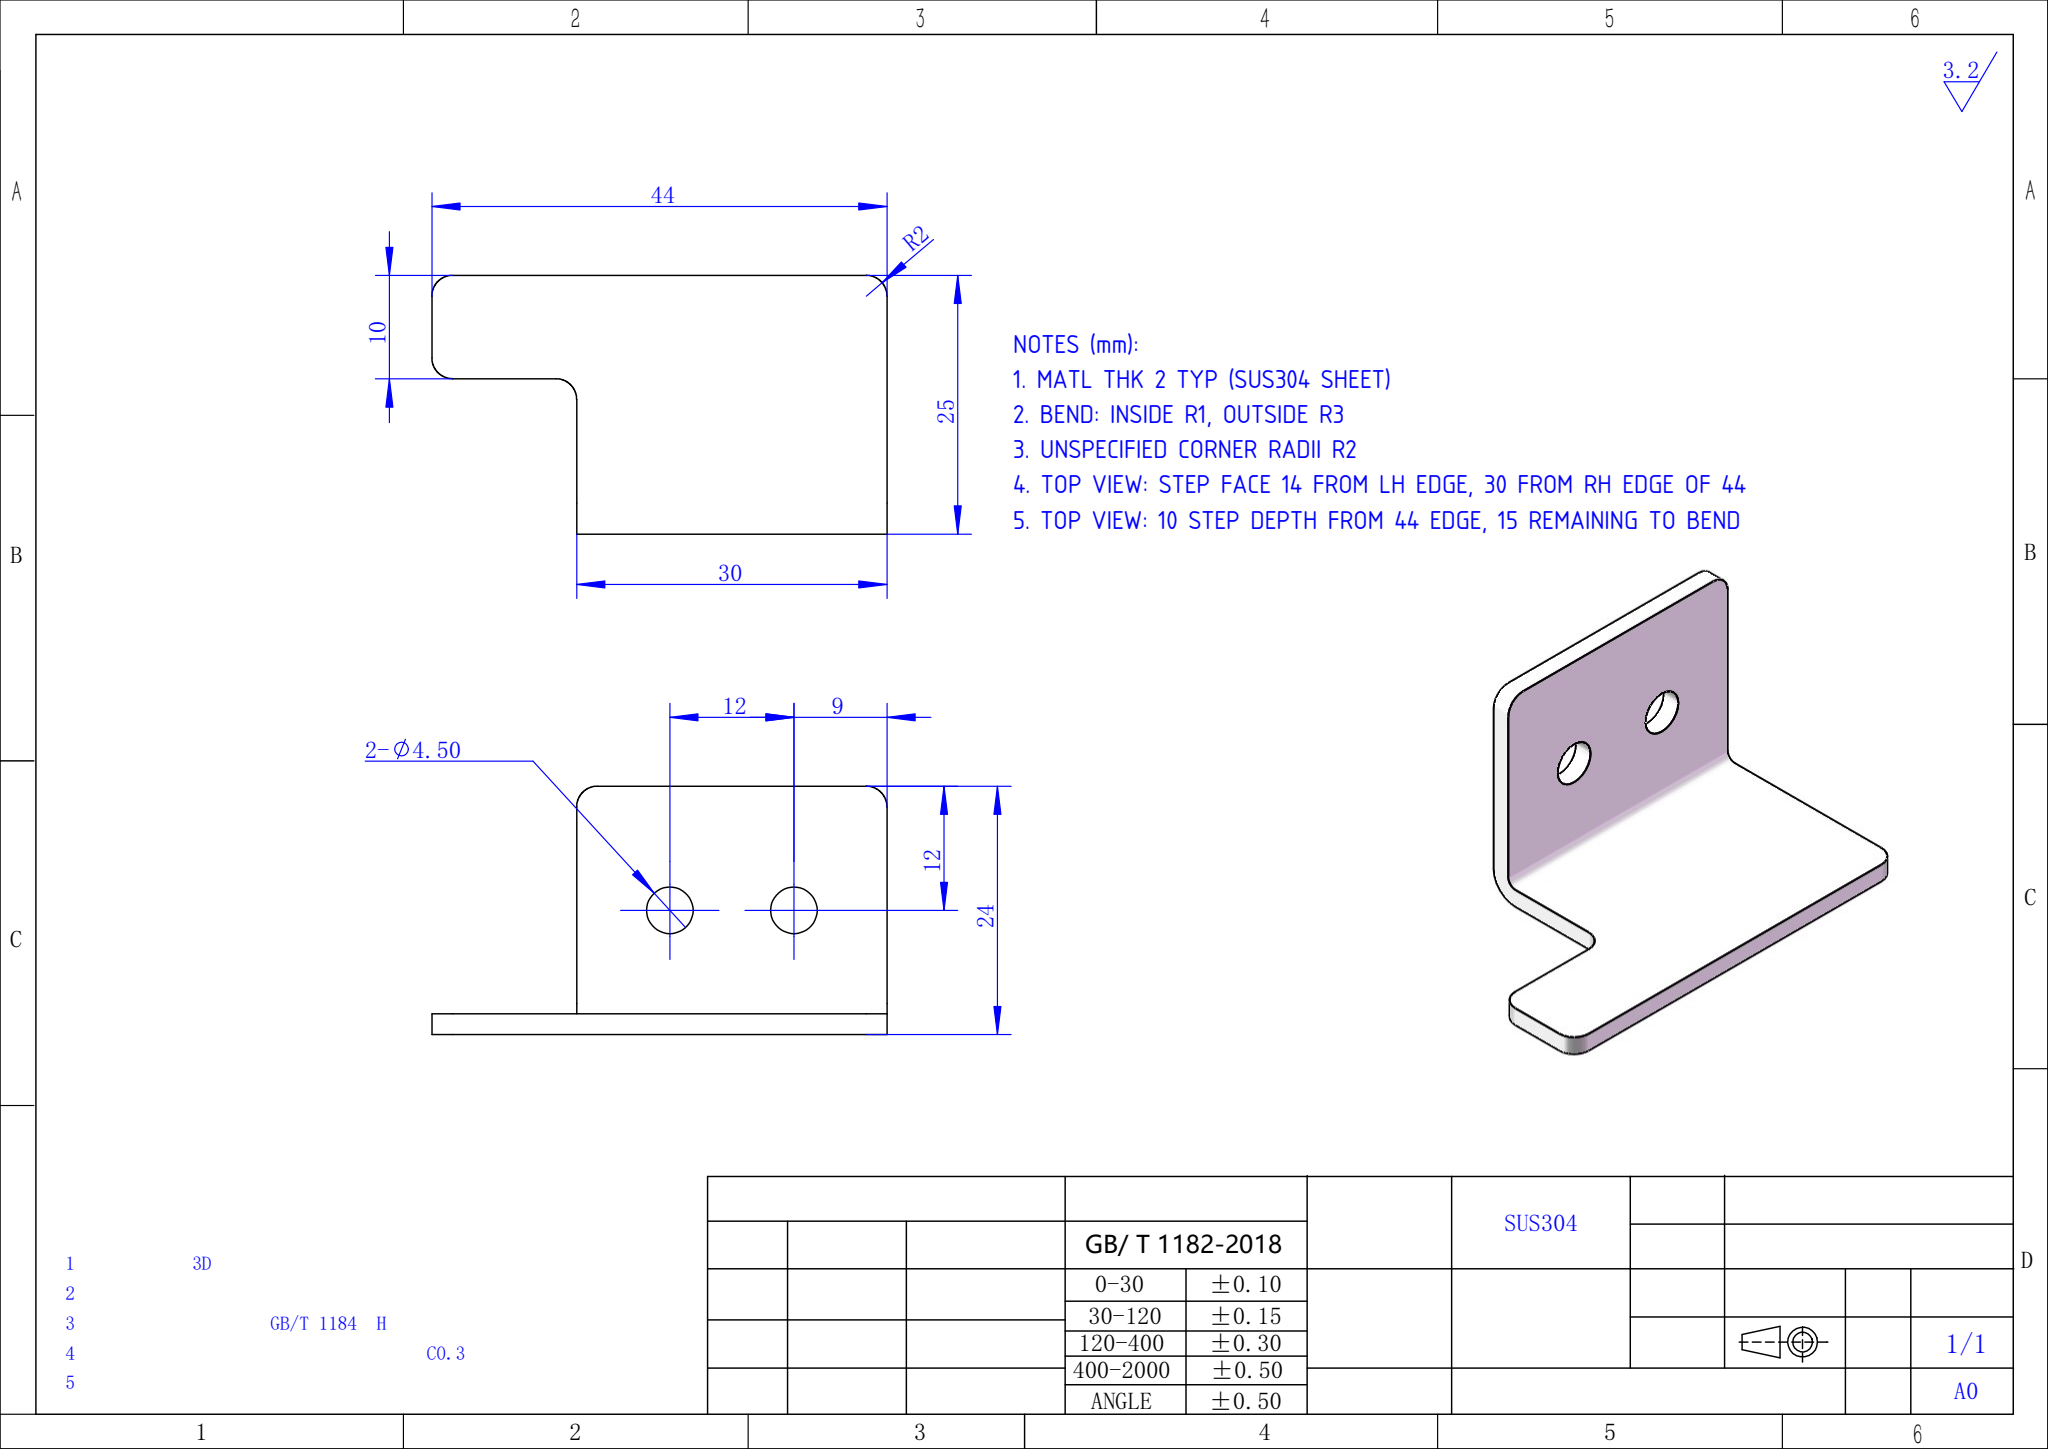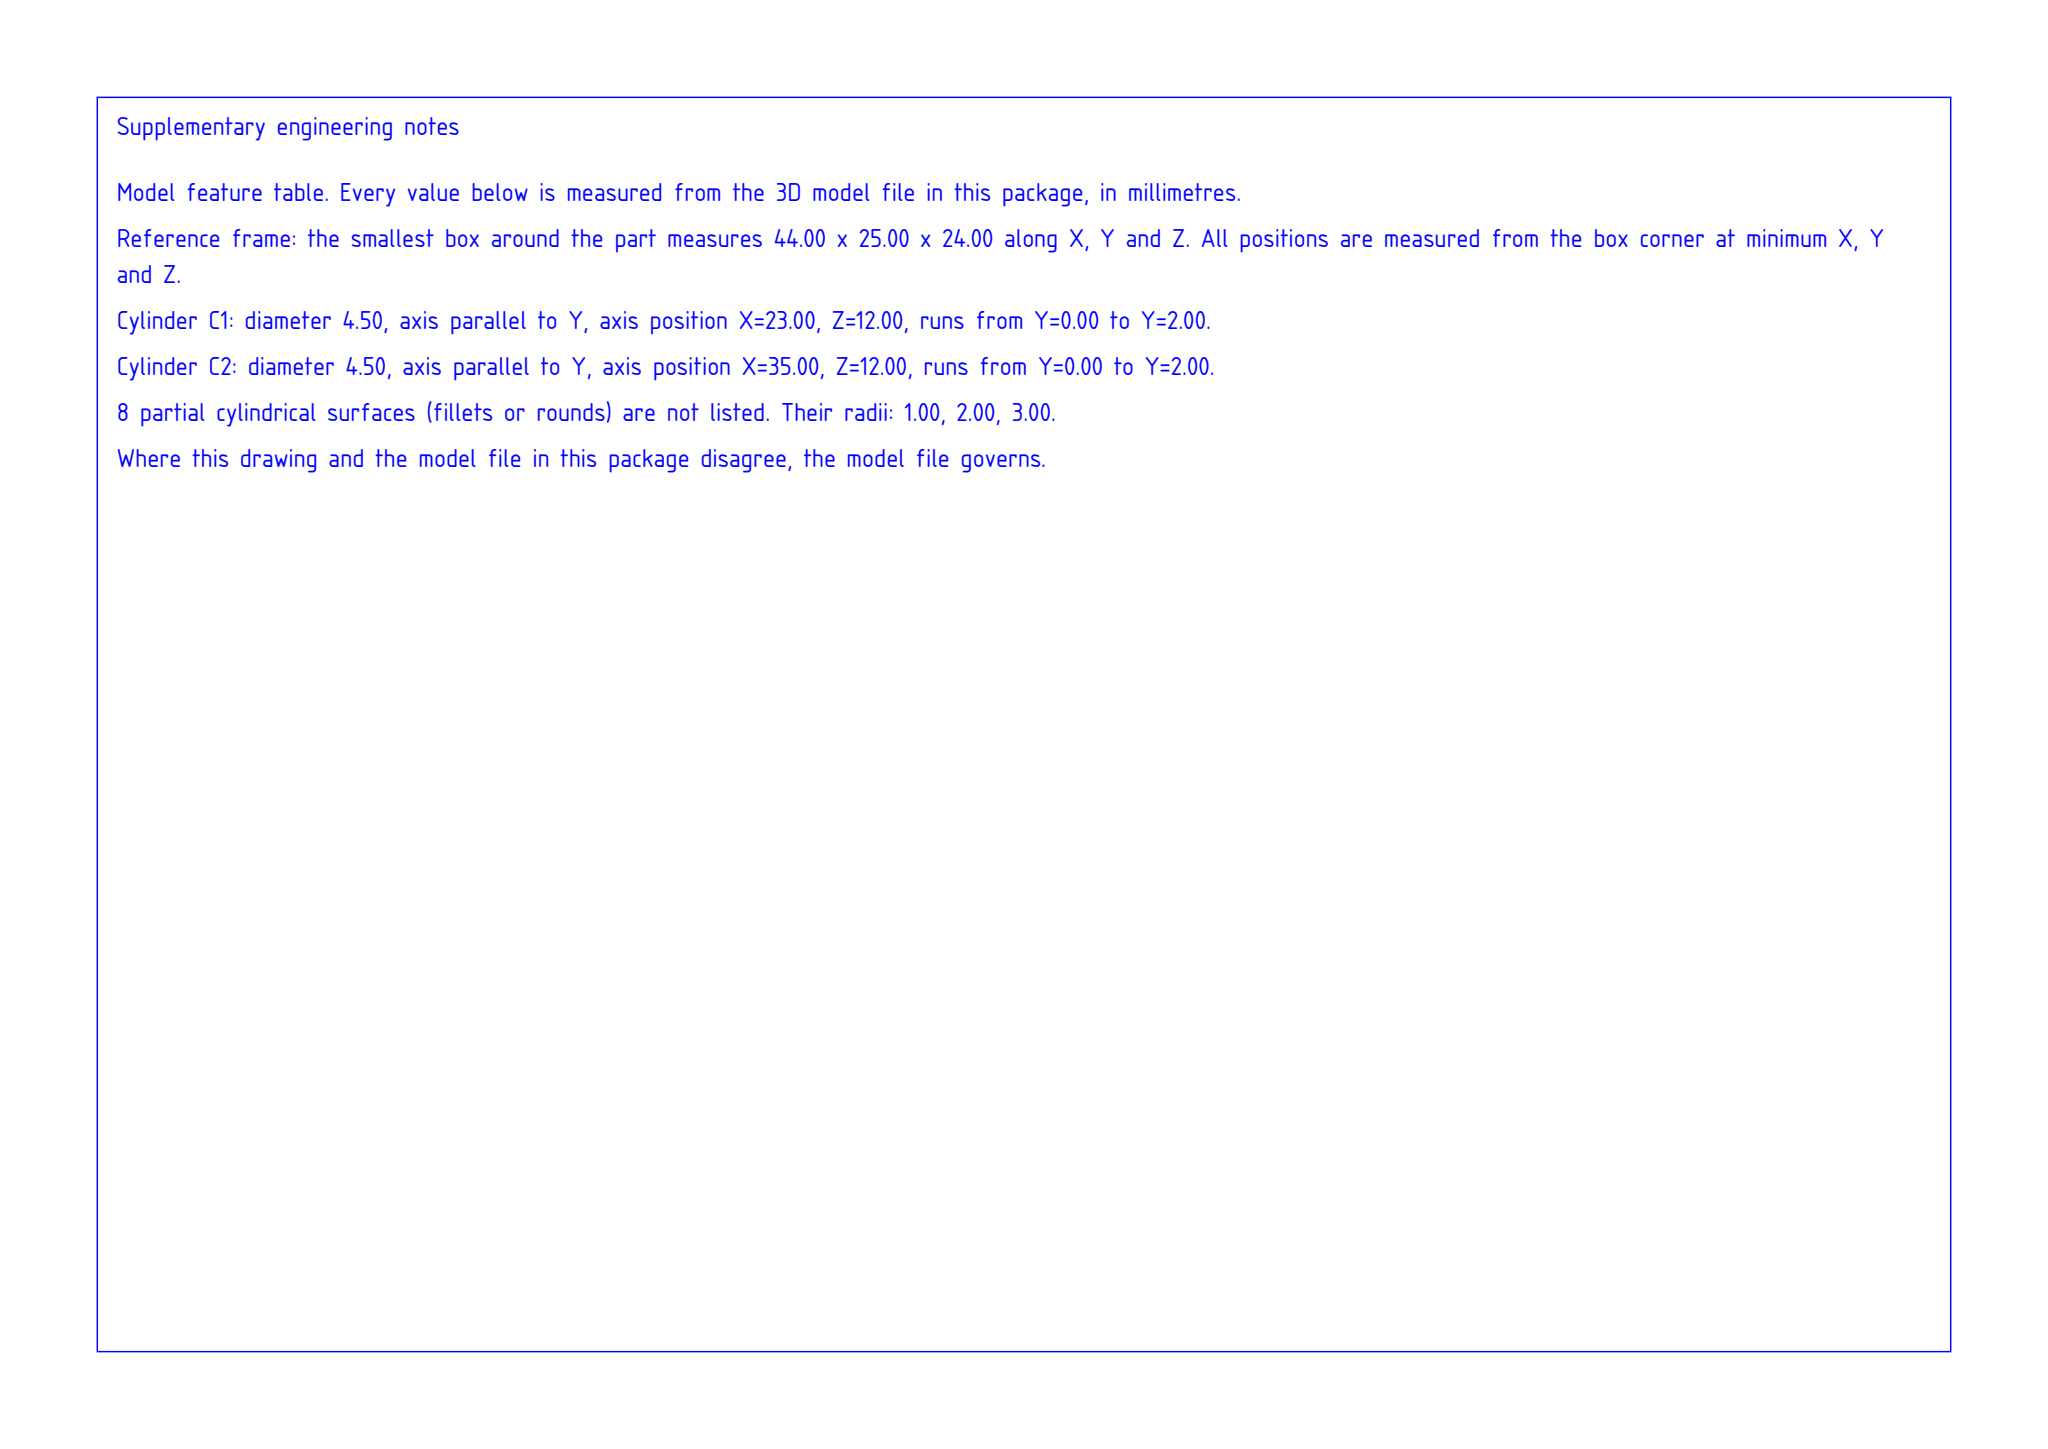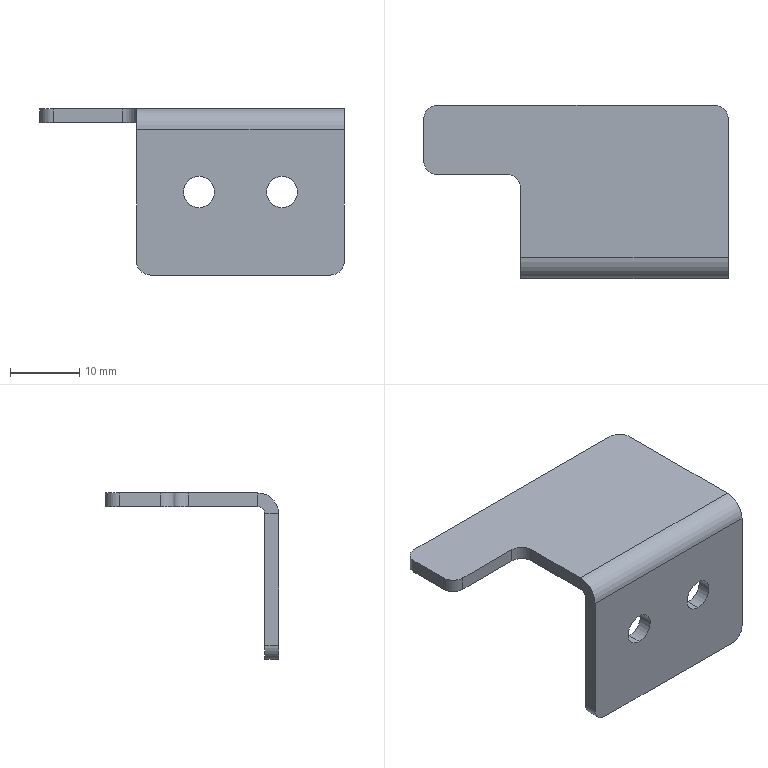Part | SolidWorks | mm | 1 solid | 26 faces | box 44 x 25 x 24 mm | volume 2978 mm3 | plane 14 | cylinder 12 | commonest cylinder face diameters 4 x6 4.5 x4 2 x1 6 x1
Drawing notes:
MATL THK 2 TYP (SUS304 SHEET) | from the solid: Y planes 0 & 2 (horiz plate), Z planes 22 & 24 (vert plate) => 2 mm wall
BEND: INSIDE R1, OUTSIDE R3 | from the solid: X-axis cyls dia 2.0 and dia 6.0 at (y=3,z=21), len 30 = bend inner/outer
UNSPECIFIED CORNER RADII R2 | from the solid: Dia 4.0 vertical/horiz corner cyls at (2,17),(2,23),(12,13),(42,23),(16,2),(42,2)
TOP VIEW: STEP FACE 14 FROM LH EDGE, 30 FROM RH EDGE OF 44 | from the solid: X plane at 14.0 (3 faces) vs bbox X 0-44; 44-14=30 matches 30 dim
TOP VIEW: 10 STEP DEPTH FROM 44 EDGE, 15 REMAINING TO BEND | from the solid: Y plane at 15.0 vs bbox Y 0-25: 25-15=10 strip, 15 remainder
STEP:
#1=CARTESIAN_POINT('',(35.,-2.,-12.25));
#2=VERTEX_POINT('',#1);
#3=CARTESIAN_POINT('',(35.,-2.,-7.75));
#4=VERTEX_POINT('',#3);
#5=CARTESIAN_POINT('',(35.,-2.,-10.));
#6=DIRECTION('',(0.,1.,0.));
#7=DIRECTION('',(0.,0.,1.));
#8=AXIS2_PLACEMENT_3D('',#5,#6,#7);
#9=CIRCLE('',#8,2.25);
#10=EDGE_CURVE('',#2,#4,#9,.T.);
#11=ORIENTED_EDGE('',*,*,#10,.F.);
#12=CARTESIAN_POINT('',(35.,-0.,-12.25));
#13=VERTEX_POINT('',#12);
#14=CARTESIAN_POINT('',(35.,0.,-12.25));
#15=DIRECTION('',(0.,1.,0.));
#16=VECTOR('',#15,1000.);
#17=LINE('',#14,#16);
#18=EDGE_CURVE('',#2,#13,#17,.T.);
#19=ORIENTED_EDGE('',*,*,#18,.T.);
#20=CARTESIAN_POINT('',(35.,-0.,-7.75));
#21=VERTEX_POINT('',#20);
#22=CARTESIAN_POINT('',(35.,-0.,-10.));
#23=DIRECTION('',(0.,1.,0.));
#24=DIRECTION('',(0.,0.,1.));
#25=AXIS2_PLACEMENT_3D('',#22,#23,#24);
#26=CIRCLE('',#25,2.25);
#27=EDGE_CURVE('',#13,#21,#26,.T.);
#28=ORIENTED_EDGE('',*,*,#27,.T.);
#29=CARTESIAN_POINT('',(35.,0.,-7.75));
#30=DIRECTION('',(0.,1.,0.));
#31=VECTOR('',#30,1000.);
#32=LINE('',#29,#31);
#33=EDGE_CURVE('',#4,#21,#32,.T.);
#34=ORIENTED_EDGE('',*,*,#33,.F.);
#35=EDGE_LOOP('',(#11,#19,#28,#34));
#36=FACE_OUTER_BOUND('',#35,.T.);
#37=CARTESIAN_POINT('',(35.,0.,-10.));
#38=DIRECTION('',(0.,1.,0.));
#39=DIRECTION('',(0.,0.,1.));
#40=AXIS2_PLACEMENT_3D('',#37,#38,#39);
#41=CYLINDRICAL_SURFACE('',#40,2.25);
#42=ADVANCED_FACE('',(#36),#41,.F.);
#43=CARTESIAN_POINT('',(23.,-2.,-12.25));
#44=VERTEX_POINT('',#43);
#45=CARTESIAN_POINT('',(23.,-2.,-7.75));
#46=VERTEX_POINT('',#45);
#47=CARTESIAN_POINT('',(23.,-2.,-10.));
#48=DIRECTION('',(0.,1.,0.));
#49=DIRECTION('',(0.,0.,1.));
#50=AXIS2_PLACEMENT_3D('',#47,#48,#49);
#51=CIRCLE('',#50,2.25);
#52=EDGE_CURVE('',#44,#46,#51,.T.);
#53=ORIENTED_EDGE('',*,*,#52,.F.);
#54=CARTESIAN_POINT('',(23.,-0.,-12.25));
#55=VERTEX_POINT('',#54);
#56=CARTESIAN_POINT('',(23.,0.,-12.25));
#57=DIRECTION('',(0.,1.,0.));
#58=VECTOR('',#57,1000.);
#59=LINE('',#56,#58);
#60=EDGE_CURVE('',#44,#55,#59,.T.);
#61=ORIENTED_EDGE('',*,*,#60,.T.);
#62=CARTESIAN_POINT('',(23.,-0.,-7.75));
#63=VERTEX_POINT('',#62);
#64=CARTESIAN_POINT('',(23.,-0.,-10.));
#65=DIRECTION('',(0.,1.,0.));
#66=DIRECTION('',(0.,0.,1.));
#67=AXIS2_PLACEMENT_3D('',#64,#65,#66);
#68=CIRCLE('',#67,2.25);
#69=EDGE_CURVE('',#55,#63,#68,.T.);
#70=ORIENTED_EDGE('',*,*,#69,.T.);
#71=CARTESIAN_POINT('',(23.,0.,-7.75));
#72=DIRECTION('',(0.,1.,0.));
#73=VECTOR('',#72,1000.);
#74=LINE('',#71,#73);
#75=EDGE_CURVE('',#46,#63,#74,.T.);
#76=ORIENTED_EDGE('',*,*,#75,.F.);
#77=EDGE_LOOP('',(#53,#61,#70,#76));
#78=FACE_OUTER_BOUND('',#77,.T.);
#79=CARTESIAN_POINT('',(23.,0.,-10.));
#80=DIRECTION('',(0.,1.,0.));
#81=DIRECTION('',(0.,0.,1.));
#82=AXIS2_PLACEMENT_3D('',#79,#80,#81);
#83=CYLINDRICAL_SURFACE('',#82,2.25);
#84=ADVANCED_FACE('',(#78),#83,.F.);
#85=CARTESIAN_POINT('',(14.,11.,2.));
#86=VERTEX_POINT('',#85);
#87=CARTESIAN_POINT('',(14.,1.,2.));
#88=VERTEX_POINT('',#87);
#89=CARTESIAN_POINT('',(14.,13.,2.));
#90=DIRECTION('',(-0.,-1.,0.));
#91=VECTOR('',#90,1000.);
#92=LINE('',#89,#91);
#93=EDGE_CURVE('',#86,#88,#92,.T.);
#94=ORIENTED_EDGE('',*,*,#93,.F.);
#95=CARTESIAN_POINT('',(14.,11.,0.));
#96=VERTEX_POINT('',#95);
#97=CARTESIAN_POINT('',(14.,11.,0.));
#98=DIRECTION('',(0.,0.,-1.));
#99=VECTOR('',#98,1000.);
#100=LINE('',#97,#99);
#101=EDGE_CURVE('',#86,#96,#100,.T.);
#102=ORIENTED_EDGE('',*,*,#101,.T.);
#103=CARTESIAN_POINT('',(14.,1.,0.));
#104=VERTEX_POINT('',#103);
#105=CARTESIAN_POINT('',(14.,0.,0.));
#106=DIRECTION('',(-0.,-1.,0.));
#107=VECTOR('',#106,1000.);
#108=LINE('',#105,#107);
#109=EDGE_CURVE('',#96,#104,#108,.T.);
#110=ORIENTED_EDGE('',*,*,#109,.T.);
#111=CARTESIAN_POINT('',(14.,1.,0.));
#112=DIRECTION('',(0.,0.,1.));
#113=VECTOR('',#112,1000.);
#114=LINE('',#111,#113);
#115=EDGE_CURVE('',#104,#88,#114,.T.);
#116=ORIENTED_EDGE('',*,*,#115,.T.);
#117=EDGE_LOOP('',(#94,#102,#110,#116));
#118=FACE_OUTER_BOUND('',#117,.T.);
#119=CARTESIAN_POINT('',(14.,13.,2.));
#120=DIRECTION('',(1.,-0.,0.));
#121=DIRECTION('',(0.,1.,0.));
#122=AXIS2_PLACEMENT_3D('',#119,#120,#121);
#123=PLANE('',#122);
#124=ADVANCED_FACE('',(#118),#123,.F.);
#125=CARTESIAN_POINT('',(14.,0.,-1.));
#126=VERTEX_POINT('',#125);
#127=CARTESIAN_POINT('',(14.,0.,-20.));
#128=VERTEX_POINT('',#127);
#129=CARTESIAN_POINT('',(14.,0.,0.));
#130=DIRECTION('',(0.,0.,-1.));
#131=VECTOR('',#130,1000.);
#132=LINE('',#129,#131);
#133=EDGE_CURVE('',#126,#128,#132,.T.);
#134=ORIENTED_EDGE('',*,*,#133,.T.);
#135=CARTESIAN_POINT('',(14.,-2.,-20.));
#136=VERTEX_POINT('',#135);
#137=CARTESIAN_POINT('',(14.,-2.,-20.));
#138=DIRECTION('',(-0.,-1.,0.));
#139=VECTOR('',#138,1000.);
#140=LINE('',#137,#139);
#141=EDGE_CURVE('',#128,#136,#140,.T.);
#142=ORIENTED_EDGE('',*,*,#141,.T.);
#143=CARTESIAN_POINT('',(14.,-2.,-1.));
#144=VERTEX_POINT('',#143);
#145=CARTESIAN_POINT('',(14.,-2.,0.));
#146=DIRECTION('',(0.,0.,-1.));
#147=VECTOR('',#146,1000.);
#148=LINE('',#145,#147);
#149=EDGE_CURVE('',#144,#136,#148,.T.);
#150=ORIENTED_EDGE('',*,*,#149,.F.);
#151=CARTESIAN_POINT('',(14.,-2.,-1.));
#152=DIRECTION('',(0.,1.,0.));
#153=VECTOR('',#152,1000.);
#154=LINE('',#151,#153);
#155=EDGE_CURVE('',#144,#126,#154,.T.);
#156=ORIENTED_EDGE('',*,*,#155,.T.);
#157=EDGE_LOOP('',(#134,#142,#150,#156));
#158=FACE_OUTER_BOUND('',#157,.T.);
#159=CARTESIAN_POINT('',(14.,13.,2.));
#160=DIRECTION('',(1.,-0.,0.));
#161=DIRECTION('',(0.,1.,0.));
#162=AXIS2_PLACEMENT_3D('',#159,#160,#161);
#163=PLANE('',#162);
#164=ADVANCED_FACE('',(#158),#163,.F.);
#165=CARTESIAN_POINT('',(44.,0.,-1.));
#166=VERTEX_POINT('',#165);
#167=CARTESIAN_POINT('',(44.,-2.,-1.));
#168=VERTEX_POINT('',#167);
#169=CARTESIAN_POINT('',(44.,0.,-1.));
#170=DIRECTION('',(0.,-1.,0.));
#171=VECTOR('',#170,1000.);
#172=LINE('',#169,#171);
#173=EDGE_CURVE('',#166,#168,#172,.T.);
#174=ORIENTED_EDGE('',*,*,#173,.F.);
#175=CARTESIAN_POINT('',(44.,1.,0.));
#176=VERTEX_POINT('',#175);
#177=CARTESIAN_POINT('',(44.,1.,-1.));
#178=DIRECTION('',(1.,0.,0.));
#179=DIRECTION('',(0.,0.,1.));
#180=AXIS2_PLACEMENT_3D('',#177,#178,#179);
#181=CIRCLE('',#180,1.);
#182=EDGE_CURVE('',#176,#166,#181,.T.);
#183=ORIENTED_EDGE('',*,*,#182,.F.);
#184=CARTESIAN_POINT('',(44.,1.,2.));
#185=VERTEX_POINT('',#184);
#186=CARTESIAN_POINT('',(44.,1.,2.));
#187=DIRECTION('',(0.,-0.,-1.));
#188=VECTOR('',#187,1000.);
#189=LINE('',#186,#188);
#190=EDGE_CURVE('',#185,#176,#189,.T.);
#191=ORIENTED_EDGE('',*,*,#190,.F.);
#192=CARTESIAN_POINT('',(44.,1.,-1.));
#193=DIRECTION('',(1.,0.,0.));
#194=DIRECTION('',(0.,0.,-1.));
#195=AXIS2_PLACEMENT_3D('',#192,#193,#194);
#196=CIRCLE('',#195,3.);
#197=EDGE_CURVE('',#185,#168,#196,.T.);
#198=ORIENTED_EDGE('',*,*,#197,.T.);
#199=EDGE_LOOP('',(#174,#183,#191,#198));
#200=FACE_OUTER_BOUND('',#199,.T.);
#201=CARTESIAN_POINT('',(44.,0.,-1.));
#202=DIRECTION('',(1.,0.,0.));
#203=DIRECTION('',(0.,0.,-1.));
#204=AXIS2_PLACEMENT_3D('',#201,#202,#203);
#205=PLANE('',#204);
#206=ADVANCED_FACE('',(#200),#205,.T.);
#207=CARTESIAN_POINT('',(44.,-2.,-20.));
#208=VERTEX_POINT('',#207);
#209=CARTESIAN_POINT('',(44.,-2.,0.));
#210=DIRECTION('',(0.,0.,-1.));
#211=VECTOR('',#210,1000.);
#212=LINE('',#209,#211);
#213=EDGE_CURVE('',#168,#208,#212,.T.);
#214=ORIENTED_EDGE('',*,*,#213,.T.);
#215=CARTESIAN_POINT('',(44.,0.,-20.));
#216=VERTEX_POINT('',#215);
#217=CARTESIAN_POINT('',(44.,1.,-20.));
#218=DIRECTION('',(0.,1.,0.));
#219=VECTOR('',#218,1000.);
#220=LINE('',#217,#219);
#221=EDGE_CURVE('',#208,#216,#220,.T.);
#222=ORIENTED_EDGE('',*,*,#221,.T.);
#223=CARTESIAN_POINT('',(44.,0.,0.));
#224=DIRECTION('',(0.,0.,-1.));
#225=VECTOR('',#224,1000.);
#226=LINE('',#223,#225);
#227=EDGE_CURVE('',#166,#216,#226,.T.);
#228=ORIENTED_EDGE('',*,*,#227,.F.);
#229=ORIENTED_EDGE('',*,*,#173,.T.);
#230=EDGE_LOOP('',(#214,#222,#228,#229));
#231=FACE_OUTER_BOUND('',#230,.T.);
#232=CARTESIAN_POINT('',(44.,1.,2.));
#233=DIRECTION('',(1.,0.,0.));
#234=DIRECTION('',(0.,0.,-1.));
#235=AXIS2_PLACEMENT_3D('',#232,#233,#234);
#236=PLANE('',#235);
#237=ADVANCED_FACE('',(#231),#236,.T.);
#238=CARTESIAN_POINT('',(0.,21.,0.));
#239=VERTEX_POINT('',#238);
#240=CARTESIAN_POINT('',(0.,15.,0.));
#241=VERTEX_POINT('',#240);
#242=CARTESIAN_POINT('',(0.,0.,0.));
#243=DIRECTION('',(0.,-1.,0.));
#244=VECTOR('',#243,1000.);
#245=LINE('',#242,#244);
#246=EDGE_CURVE('',#239,#241,#245,.T.);
#247=ORIENTED_EDGE('',*,*,#246,.T.);
#248=CARTESIAN_POINT('',(0.,15.,2.));
#249=VERTEX_POINT('',#248);
#250=CARTESIAN_POINT('',(0.,15.,2.));
#251=DIRECTION('',(0.,0.,1.));
#252=VECTOR('',#251,1000.);
#253=LINE('',#250,#252);
#254=EDGE_CURVE('',#241,#249,#253,.T.);
#255=ORIENTED_EDGE('',*,*,#254,.T.);
#256=CARTESIAN_POINT('',(0.,21.,2.));
#257=VERTEX_POINT('',#256);
#258=CARTESIAN_POINT('',(0.,0.,2.));
#259=DIRECTION('',(0.,-1.,0.));
#260=VECTOR('',#259,1000.);
#261=LINE('',#258,#260);
#262=EDGE_CURVE('',#257,#249,#261,.T.);
#263=ORIENTED_EDGE('',*,*,#262,.F.);
#264=CARTESIAN_POINT('',(0.,21.,-1.));
#265=DIRECTION('',(0.,0.,-1.));
#266=VECTOR('',#265,1000.);
#267=LINE('',#264,#266);
#268=EDGE_CURVE('',#257,#239,#267,.T.);
#269=ORIENTED_EDGE('',*,*,#268,.T.);
#270=EDGE_LOOP('',(#247,#255,#263,#269));
#271=FACE_OUTER_BOUND('',#270,.T.);
#272=CARTESIAN_POINT('',(0.,-2.,-1.));
#273=DIRECTION('',(-1.,0.,0.));
#274=DIRECTION('',(0.,0.,1.));
#275=AXIS2_PLACEMENT_3D('',#272,#273,#274);
#276=PLANE('',#275);
#277=ADVANCED_FACE('',(#271),#276,.T.);
#278=CARTESIAN_POINT('',(35.,-2.,-10.));
#279=DIRECTION('',(0.,1.,0.));
#280=DIRECTION('',(0.,0.,1.));
#281=AXIS2_PLACEMENT_3D('',#278,#279,#280);
#282=CIRCLE('',#281,2.25);
#283=EDGE_CURVE('',#4,#2,#282,.T.);
#284=ORIENTED_EDGE('',*,*,#283,.T.);
#285=ORIENTED_EDGE('',*,*,#10,.T.);
#286=EDGE_LOOP('',(#284,#285));
#287=FACE_BOUND('',#286,.T.);
#288=CARTESIAN_POINT('',(23.,-2.,-10.));
#289=DIRECTION('',(0.,1.,0.));
#290=DIRECTION('',(0.,0.,1.));
#291=AXIS2_PLACEMENT_3D('',#288,#289,#290);
#292=CIRCLE('',#291,2.25);
#293=EDGE_CURVE('',#46,#44,#292,.T.);
#294=ORIENTED_EDGE('',*,*,#293,.T.);
#295=ORIENTED_EDGE('',*,*,#52,.T.);
#296=EDGE_LOOP('',(#294,#295));
#297=FACE_BOUND('',#296,.T.);
#298=CARTESIAN_POINT('',(42.,-2.,-22.));
#299=VERTEX_POINT('',#298);
#300=CARTESIAN_POINT('',(16.,-2.,-22.));
#301=VERTEX_POINT('',#300);
#302=CARTESIAN_POINT('',(44.,-2.,-22.));
#303=DIRECTION('',(-1.,0.,0.));
#304=VECTOR('',#303,1000.);
#305=LINE('',#302,#304);
#306=EDGE_CURVE('',#299,#301,#305,.T.);
#307=ORIENTED_EDGE('',*,*,#306,.F.);
#308=CARTESIAN_POINT('',(42.,-2.,-20.));
#309=DIRECTION('',(0.,-1.,0.));
#310=DIRECTION('',(0.,0.,1.));
#311=AXIS2_PLACEMENT_3D('',#308,#309,#310);
#312=CIRCLE('',#311,2.);
#313=EDGE_CURVE('',#299,#208,#312,.T.);
#314=ORIENTED_EDGE('',*,*,#313,.T.);
#315=ORIENTED_EDGE('',*,*,#213,.F.);
#316=CARTESIAN_POINT('',(44.,-2.,-1.));
#317=DIRECTION('',(-1.,0.,0.));
#318=VECTOR('',#317,1000.);
#319=LINE('',#316,#318);
#320=EDGE_CURVE('',#168,#144,#319,.T.);
#321=ORIENTED_EDGE('',*,*,#320,.T.);
#322=ORIENTED_EDGE('',*,*,#149,.T.);
#323=CARTESIAN_POINT('',(16.,-2.,-20.));
#324=DIRECTION('',(0.,-1.,0.));
#325=DIRECTION('',(0.,0.,1.));
#326=AXIS2_PLACEMENT_3D('',#323,#324,#325);
#327=CIRCLE('',#326,2.);
#328=EDGE_CURVE('',#136,#301,#327,.T.);
#329=ORIENTED_EDGE('',*,*,#328,.T.);
#330=EDGE_LOOP('',(#307,#314,#315,#321,#322,#329));
#331=FACE_OUTER_BOUND('',#330,.T.);
#332=CARTESIAN_POINT('',(44.,-2.,0.));
#333=DIRECTION('',(0.,1.,0.));
#334=DIRECTION('',(0.,0.,1.));
#335=AXIS2_PLACEMENT_3D('',#332,#333,#334);
#336=PLANE('',#335);
#337=ADVANCED_FACE('',(#287,#297,#331),#336,.F.);
#338=CARTESIAN_POINT('',(42.,0.,-22.));
#339=VERTEX_POINT('',#338);
#340=CARTESIAN_POINT('',(16.,0.,-22.));
#341=VERTEX_POINT('',#340);
#342=CARTESIAN_POINT('',(44.,0.,-22.));
#343=DIRECTION('',(-1.,0.,0.));
#344=VECTOR('',#343,1000.);
#345=LINE('',#342,#344);
#346=EDGE_CURVE('',#339,#341,#345,.T.);
#347=ORIENTED_EDGE('',*,*,#346,.F.);
#348=CARTESIAN_POINT('',(42.,0.,-22.));
#349=DIRECTION('',(0.,-1.,0.));
#350=VECTOR('',#349,1000.);
#351=LINE('',#348,#350);
#352=EDGE_CURVE('',#339,#299,#351,.T.);
#353=ORIENTED_EDGE('',*,*,#352,.T.);
#354=ORIENTED_EDGE('',*,*,#306,.T.);
#355=CARTESIAN_POINT('',(16.,0.,-22.));
#356=DIRECTION('',(0.,1.,0.));
#357=VECTOR('',#356,1000.);
#358=LINE('',#355,#357);
#359=EDGE_CURVE('',#301,#341,#358,.T.);
#360=ORIENTED_EDGE('',*,*,#359,.T.);
#361=EDGE_LOOP('',(#347,#353,#354,#360));
#362=FACE_OUTER_BOUND('',#361,.T.);
#363=CARTESIAN_POINT('',(44.,0.,-22.));
#364=DIRECTION('',(0.,0.,-1.));
#365=DIRECTION('',(-1.,0.,0.));
#366=AXIS2_PLACEMENT_3D('',#363,#364,#365);
#367=PLANE('',#366);
#368=ADVANCED_FACE('',(#362),#367,.T.);
#369=CARTESIAN_POINT('',(35.,-0.,-10.));
#370=DIRECTION('',(0.,1.,0.));
#371=DIRECTION('',(0.,0.,1.));
#372=AXIS2_PLACEMENT_3D('',#369,#370,#371);
#373=CIRCLE('',#372,2.25);
#374=EDGE_CURVE('',#21,#13,#373,.T.);
#375=ORIENTED_EDGE('',*,*,#374,.F.);
#376=ORIENTED_EDGE('',*,*,#27,.F.);
#377=EDGE_LOOP('',(#375,#376));
#378=FACE_BOUND('',#377,.T.);
#379=CARTESIAN_POINT('',(23.,-0.,-10.));
#380=DIRECTION('',(0.,1.,0.));
#381=DIRECTION('',(0.,0.,1.));
#382=AXIS2_PLACEMENT_3D('',#379,#380,#381);
#383=CIRCLE('',#382,2.25);
#384=EDGE_CURVE('',#63,#55,#383,.T.);
#385=ORIENTED_EDGE('',*,*,#384,.F.);
#386=ORIENTED_EDGE('',*,*,#69,.F.);
#387=EDGE_LOOP('',(#385,#386));
#388=FACE_BOUND('',#387,.T.);
#389=ORIENTED_EDGE('',*,*,#227,.T.);
#390=CARTESIAN_POINT('',(42.,0.,-20.));
#391=DIRECTION('',(0.,1.,0.));
#392=DIRECTION('',(0.,0.,1.));
#393=AXIS2_PLACEMENT_3D('',#390,#391,#392);
#394=CIRCLE('',#393,2.);
#395=EDGE_CURVE('',#216,#339,#394,.T.);
#396=ORIENTED_EDGE('',*,*,#395,.T.);
#397=ORIENTED_EDGE('',*,*,#346,.T.);
#398=CARTESIAN_POINT('',(16.,0.,-20.));
#399=DIRECTION('',(0.,1.,0.));
#400=DIRECTION('',(0.,0.,1.));
#401=AXIS2_PLACEMENT_3D('',#398,#399,#400);
#402=CIRCLE('',#401,2.);
#403=EDGE_CURVE('',#341,#128,#402,.T.);
#404=ORIENTED_EDGE('',*,*,#403,.T.);
#405=ORIENTED_EDGE('',*,*,#133,.F.);
#406=CARTESIAN_POINT('',(44.,0.,-1.));
#407=DIRECTION('',(-1.,0.,0.));
#408=VECTOR('',#407,1000.);
#409=LINE('',#406,#408);
#410=EDGE_CURVE('',#166,#126,#409,.T.);
#411=ORIENTED_EDGE('',*,*,#410,.F.);
#412=EDGE_LOOP('',(#389,#396,#397,#404,#405,#411));
#413=FACE_OUTER_BOUND('',#412,.T.);
#414=CARTESIAN_POINT('',(44.,0.,0.));
#415=DIRECTION('',(0.,1.,0.));
#416=DIRECTION('',(0.,0.,1.));
#417=AXIS2_PLACEMENT_3D('',#414,#415,#416);
#418=PLANE('',#417);
#419=ADVANCED_FACE('',(#378,#388,#413),#418,.T.);
#420=CARTESIAN_POINT('',(14.,1.,-1.));
#421=DIRECTION('',(1.,-0.,0.));
#422=DIRECTION('',(0.,1.,0.));
#423=AXIS2_PLACEMENT_3D('',#420,#421,#422);
#424=CIRCLE('',#423,1.);
#425=EDGE_CURVE('',#104,#126,#424,.T.);
#426=ORIENTED_EDGE('',*,*,#425,.F.);
#427=CARTESIAN_POINT('',(44.,1.,0.));
#428=DIRECTION('',(-1.,0.,0.));
#429=VECTOR('',#428,1000.);
#430=LINE('',#427,#429);
#431=EDGE_CURVE('',#176,#104,#430,.T.);
#432=ORIENTED_EDGE('',*,*,#431,.F.);
#433=ORIENTED_EDGE('',*,*,#182,.T.);
#434=ORIENTED_EDGE('',*,*,#410,.T.);
#435=EDGE_LOOP('',(#426,#432,#433,#434));
#436=FACE_OUTER_BOUND('',#435,.T.);
#437=CARTESIAN_POINT('',(44.,1.,-1.));
#438=DIRECTION('',(-1.,0.,0.));
#439=DIRECTION('',(0.,0.,1.));
#440=AXIS2_PLACEMENT_3D('',#437,#438,#439);
#441=CYLINDRICAL_SURFACE('',#440,1.);
#442=ADVANCED_FACE('',(#436),#441,.F.);
#443=CARTESIAN_POINT('',(2.,13.,0.));
#444=VERTEX_POINT('',#443);
#445=CARTESIAN_POINT('',(12.,13.,0.));
#446=VERTEX_POINT('',#445);
#447=CARTESIAN_POINT('',(44.,13.,0.));
#448=DIRECTION('',(1.,0.,0.));
#449=VECTOR('',#448,1000.);
#450=LINE('',#447,#449);
#451=EDGE_CURVE('',#444,#446,#450,.T.);
#452=ORIENTED_EDGE('',*,*,#451,.F.);
#453=CARTESIAN_POINT('',(2.,15.,0.));
#454=DIRECTION('',(0.,0.,-1.));
#455=DIRECTION('',(-1.,0.,0.));
#456=AXIS2_PLACEMENT_3D('',#453,#454,#455);
#457=CIRCLE('',#456,2.);
#458=EDGE_CURVE('',#444,#241,#457,.T.);
#459=ORIENTED_EDGE('',*,*,#458,.T.);
#460=ORIENTED_EDGE('',*,*,#246,.F.);
#461=CARTESIAN_POINT('',(2.,23.,0.));
#462=VERTEX_POINT('',#461);
#463=CARTESIAN_POINT('',(2.,21.,0.));
#464=DIRECTION('',(0.,0.,-1.));
#465=DIRECTION('',(-1.,0.,0.));
#466=AXIS2_PLACEMENT_3D('',#463,#464,#465);
#467=CIRCLE('',#466,2.);
#468=EDGE_CURVE('',#239,#462,#467,.T.);
#469=ORIENTED_EDGE('',*,*,#468,.T.);
#470=CARTESIAN_POINT('',(42.,23.,0.));
#471=VERTEX_POINT('',#470);
#472=CARTESIAN_POINT('',(44.,23.,0.));
#473=DIRECTION('',(-1.,0.,0.));
#474=VECTOR('',#473,1000.);
#475=LINE('',#472,#474);
#476=EDGE_CURVE('',#471,#462,#475,.T.);
#477=ORIENTED_EDGE('',*,*,#476,.F.);
#478=CARTESIAN_POINT('',(44.,21.,0.));
#479=VERTEX_POINT('',#478);
#480=CARTESIAN_POINT('',(42.,21.,0.));
#481=DIRECTION('',(0.,0.,-1.));
#482=DIRECTION('',(-1.,0.,0.));
#483=AXIS2_PLACEMENT_3D('',#480,#481,#482);
#484=CIRCLE('',#483,2.);
#485=EDGE_CURVE('',#471,#479,#484,.T.);
#486=ORIENTED_EDGE('',*,*,#485,.T.);
#487=CARTESIAN_POINT('',(44.,0.,0.));
#488=DIRECTION('',(0.,-1.,0.));
#489=VECTOR('',#488,1000.);
#490=LINE('',#487,#489);
#491=EDGE_CURVE('',#479,#176,#490,.T.);
#492=ORIENTED_EDGE('',*,*,#491,.T.);
#493=ORIENTED_EDGE('',*,*,#431,.T.);
#494=ORIENTED_EDGE('',*,*,#109,.F.);
#495=CARTESIAN_POINT('',(12.,11.,0.));
#496=DIRECTION('',(0.,0.,1.));
#497=DIRECTION('',(-1.,0.,0.));
#498=AXIS2_PLACEMENT_3D('',#495,#496,#497);
#499=CIRCLE('',#498,2.);
#500=EDGE_CURVE('',#96,#446,#499,.T.);
#501=ORIENTED_EDGE('',*,*,#500,.T.);
#502=EDGE_LOOP('',(#452,#459,#460,#469,#477,#486,#492,#493,#494,#501));
#503=FACE_OUTER_BOUND('',#502,.T.);
#504=CARTESIAN_POINT('',(44.,0.,0.));
#505=DIRECTION('',(0.,0.,-1.));
#506=DIRECTION('',(-1.,0.,0.));
#507=AXIS2_PLACEMENT_3D('',#504,#505,#506);
#508=PLANE('',#507);
#509=ADVANCED_FACE('',(#503),#508,.T.);
#510=ORIENTED_EDGE('',*,*,#476,.T.);
#511=CARTESIAN_POINT('',(2.,23.,2.));
#512=VERTEX_POINT('',#511);
#513=CARTESIAN_POINT('',(2.,23.,2.));
#514=DIRECTION('',(0.,0.,1.));
#515=VECTOR('',#514,1000.);
#516=LINE('',#513,#515);
#517=EDGE_CURVE('',#462,#512,#516,.T.);
#518=ORIENTED_EDGE('',*,*,#517,.T.);
#519=CARTESIAN_POINT('',(42.,23.,2.));
#520=VERTEX_POINT('',#519);
#521=CARTESIAN_POINT('',(44.,23.,2.));
#522=DIRECTION('',(-1.,0.,0.));
#523=VECTOR('',#522,1000.);
#524=LINE('',#521,#523);
#525=EDGE_CURVE('',#520,#512,#524,.T.);
#526=ORIENTED_EDGE('',*,*,#525,.F.);
#527=CARTESIAN_POINT('',(42.,23.,0.));
#528=DIRECTION('',(0.,0.,-1.));
#529=VECTOR('',#528,1000.);
#530=LINE('',#527,#529);
#531=EDGE_CURVE('',#520,#471,#530,.T.);
#532=ORIENTED_EDGE('',*,*,#531,.T.);
#533=EDGE_LOOP('',(#510,#518,#526,#532));
#534=FACE_OUTER_BOUND('',#533,.T.);
#535=CARTESIAN_POINT('',(44.,23.,2.));
#536=DIRECTION('',(0.,1.,0.));
#537=DIRECTION('',(0.,0.,1.));
#538=AXIS2_PLACEMENT_3D('',#535,#536,#537);
#539=PLANE('',#538);
#540=ADVANCED_FACE('',(#534),#539,.T.);
#541=ORIENTED_EDGE('',*,*,#262,.T.);
#542=CARTESIAN_POINT('',(2.,13.,2.));
#543=VERTEX_POINT('',#542);
#544=CARTESIAN_POINT('',(2.,15.,2.));
#545=DIRECTION('',(0.,0.,1.));
#546=DIRECTION('',(-1.,0.,0.));
#547=AXIS2_PLACEMENT_3D('',#544,#545,#546);
#548=CIRCLE('',#547,2.);
#549=EDGE_CURVE('',#249,#543,#548,.T.);
#550=ORIENTED_EDGE('',*,*,#549,.T.);
#551=CARTESIAN_POINT('',(12.,13.,2.));
#552=VERTEX_POINT('',#551);
#553=CARTESIAN_POINT('',(14.,13.,2.));
#554=DIRECTION('',(1.,0.,0.));
#555=VECTOR('',#554,1000.);
#556=LINE('',#553,#555);
#557=EDGE_CURVE('',#543,#552,#556,.T.);
#558=ORIENTED_EDGE('',*,*,#557,.T.);
#559=CARTESIAN_POINT('',(12.,11.,2.));
#560=DIRECTION('',(0.,0.,-1.));
#561=DIRECTION('',(-1.,0.,0.));
#562=AXIS2_PLACEMENT_3D('',#559,#560,#561);
#563=CIRCLE('',#562,2.);
#564=EDGE_CURVE('',#552,#86,#563,.T.);
#565=ORIENTED_EDGE('',*,*,#564,.T.);
#566=ORIENTED_EDGE('',*,*,#93,.T.);
#567=CARTESIAN_POINT('',(44.,1.,2.));
#568=DIRECTION('',(-1.,0.,0.));
#569=VECTOR('',#568,1000.);
#570=LINE('',#567,#569);
#571=EDGE_CURVE('',#185,#88,#570,.T.);
#572=ORIENTED_EDGE('',*,*,#571,.F.);
#573=CARTESIAN_POINT('',(44.,21.,2.));
#574=VERTEX_POINT('',#573);
#575=CARTESIAN_POINT('',(44.,0.,2.));
#576=DIRECTION('',(0.,-1.,0.));
#577=VECTOR('',#576,1000.);
#578=LINE('',#575,#577);
#579=EDGE_CURVE('',#574,#185,#578,.T.);
#580=ORIENTED_EDGE('',*,*,#579,.F.);
#581=CARTESIAN_POINT('',(42.,21.,2.));
#582=DIRECTION('',(0.,0.,1.));
#583=DIRECTION('',(-1.,0.,0.));
#584=AXIS2_PLACEMENT_3D('',#581,#582,#583);
#585=CIRCLE('',#584,2.);
#586=EDGE_CURVE('',#574,#520,#585,.T.);
#587=ORIENTED_EDGE('',*,*,#586,.T.);
#588=ORIENTED_EDGE('',*,*,#525,.T.);
#589=CARTESIAN_POINT('',(2.,21.,2.));
#590=DIRECTION('',(0.,0.,1.));
#591=DIRECTION('',(-1.,0.,0.));
#592=AXIS2_PLACEMENT_3D('',#589,#590,#591);
#593=CIRCLE('',#592,2.);
#594=EDGE_CURVE('',#512,#257,#593,.T.);
#595=ORIENTED_EDGE('',*,*,#594,.T.);
#596=EDGE_LOOP('',(#541,#550,#558,#565,#566,#572,#580,#587,#588,#595));
#597=FACE_OUTER_BOUND('',#596,.T.);
#598=CARTESIAN_POINT('',(44.,0.,2.));
#599=DIRECTION('',(0.,0.,-1.));
#600=DIRECTION('',(-1.,0.,0.));
#601=AXIS2_PLACEMENT_3D('',#598,#599,#600);
#602=PLANE('',#601);
#603=ADVANCED_FACE('',(#597),#602,.F.);
#604=ORIENTED_EDGE('',*,*,#571,.T.);
#605=CARTESIAN_POINT('',(14.,1.,-1.));
#606=DIRECTION('',(1.,-0.,0.));
#607=DIRECTION('',(0.,1.,0.));
#608=AXIS2_PLACEMENT_3D('',#605,#606,#607);
#609=CIRCLE('',#608,3.);
#610=EDGE_CURVE('',#88,#144,#609,.T.);
#611=ORIENTED_EDGE('',*,*,#610,.T.);
#612=ORIENTED_EDGE('',*,*,#320,.F.);
#613=ORIENTED_EDGE('',*,*,#197,.F.);
#614=EDGE_LOOP('',(#604,#611,#612,#613));
#615=FACE_OUTER_BOUND('',#614,.T.);
#616=CARTESIAN_POINT('',(44.,1.,-1.));
#617=DIRECTION('',(-1.,0.,0.));
#618=DIRECTION('',(0.,0.,1.));
#619=AXIS2_PLACEMENT_3D('',#616,#617,#618);
#620=CYLINDRICAL_SURFACE('',#619,3.);
#621=ADVANCED_FACE('',(#615),#620,.T.);
#622=ORIENTED_EDGE('',*,*,#491,.F.);
#623=CARTESIAN_POINT('',(44.,21.,2.));
#624=DIRECTION('',(0.,0.,1.));
#625=VECTOR('',#624,1000.);
#626=LINE('',#623,#625);
#627=EDGE_CURVE('',#479,#574,#626,.T.);
#628=ORIENTED_EDGE('',*,*,#627,.T.);
#629=ORIENTED_EDGE('',*,*,#579,.T.);
#630=ORIENTED_EDGE('',*,*,#190,.T.);
#631=EDGE_LOOP('',(#622,#628,#629,#630));
#632=FACE_OUTER_BOUND('',#631,.T.);
#633=CARTESIAN_POINT('',(44.,1.,-1.));
#634=DIRECTION('',(-1.,0.,0.));
#635=DIRECTION('',(0.,0.,1.));
#636=AXIS2_PLACEMENT_3D('',#633,#634,#635);
#637=PLANE('',#636);
#638=ADVANCED_FACE('',(#632),#637,.F.);
#639=ORIENTED_EDGE('',*,*,#115,.F.);
#640=ORIENTED_EDGE('',*,*,#425,.T.);
#641=ORIENTED_EDGE('',*,*,#155,.F.);
#642=ORIENTED_EDGE('',*,*,#610,.F.);
#643=EDGE_LOOP('',(#639,#640,#641,#642));
#644=FACE_OUTER_BOUND('',#643,.T.);
#645=CARTESIAN_POINT('',(14.,13.,2.));
#646=DIRECTION('',(1.,-0.,0.));
#647=DIRECTION('',(0.,1.,0.));
#648=AXIS2_PLACEMENT_3D('',#645,#646,#647);
#649=PLANE('',#648);
#650=ADVANCED_FACE('',(#644),#649,.F.);
#651=ORIENTED_EDGE('',*,*,#451,.T.);
#652=CARTESIAN_POINT('',(12.,13.,2.));
#653=DIRECTION('',(0.,0.,1.));
#654=VECTOR('',#653,1000.);
#655=LINE('',#652,#654);
#656=EDGE_CURVE('',#446,#552,#655,.T.);
#657=ORIENTED_EDGE('',*,*,#656,.T.);
#658=ORIENTED_EDGE('',*,*,#557,.F.);
#659=CARTESIAN_POINT('',(2.,13.,0.));
#660=DIRECTION('',(0.,0.,-1.));
#661=VECTOR('',#660,1000.);
#662=LINE('',#659,#661);
#663=EDGE_CURVE('',#543,#444,#662,.T.);
#664=ORIENTED_EDGE('',*,*,#663,.T.);
#665=EDGE_LOOP('',(#651,#657,#658,#664));
#666=FACE_OUTER_BOUND('',#665,.T.);
#667=CARTESIAN_POINT('',(14.,13.,2.));
#668=DIRECTION('',(0.,1.,0.));
#669=DIRECTION('',(0.,0.,1.));
#670=AXIS2_PLACEMENT_3D('',#667,#668,#669);
#671=PLANE('',#670);
#672=ADVANCED_FACE('',(#666),#671,.F.);
#673=ORIENTED_EDGE('',*,*,#564,.F.);
#674=ORIENTED_EDGE('',*,*,#656,.F.);
#675=ORIENTED_EDGE('',*,*,#500,.F.);
#676=ORIENTED_EDGE('',*,*,#101,.F.);
#677=EDGE_LOOP('',(#673,#674,#675,#676));
#678=FACE_OUTER_BOUND('',#677,.T.);
#679=CARTESIAN_POINT('',(12.,11.,2.));
#680=DIRECTION('',(0.,0.,1.));
#681=DIRECTION('',(1.,0.,0.));
#682=AXIS2_PLACEMENT_3D('',#679,#680,#681);
#683=CYLINDRICAL_SURFACE('',#682,2.);
#684=ADVANCED_FACE('',(#678),#683,.F.);
#685=ORIENTED_EDGE('',*,*,#395,.F.);
#686=ORIENTED_EDGE('',*,*,#221,.F.);
#687=ORIENTED_EDGE('',*,*,#313,.F.);
#688=ORIENTED_EDGE('',*,*,#352,.F.);
#689=EDGE_LOOP('',(#685,#686,#687,#688));
#690=FACE_OUTER_BOUND('',#689,.T.);
#691=CARTESIAN_POINT('',(42.,0.,-20.));
#692=DIRECTION('',(0.,-1.,0.));
#693=DIRECTION('',(0.,0.,-1.));
#694=AXIS2_PLACEMENT_3D('',#691,#692,#693);
#695=CYLINDRICAL_SURFACE('',#694,2.);
#696=ADVANCED_FACE('',(#690),#695,.T.);
#697=ORIENTED_EDGE('',*,*,#403,.F.);
#698=ORIENTED_EDGE('',*,*,#359,.F.);
#699=ORIENTED_EDGE('',*,*,#328,.F.);
#700=ORIENTED_EDGE('',*,*,#141,.F.);
#701=EDGE_LOOP('',(#697,#698,#699,#700));
#702=FACE_OUTER_BOUND('',#701,.T.);
#703=CARTESIAN_POINT('',(16.,13.,-20.));
#704=DIRECTION('',(0.,1.,0.));
#705=DIRECTION('',(-1.,0.,0.));
#706=AXIS2_PLACEMENT_3D('',#703,#704,#705);
#707=CYLINDRICAL_SURFACE('',#706,2.);
#708=ADVANCED_FACE('',(#702),#707,.T.);
#709=ORIENTED_EDGE('',*,*,#549,.F.);
#710=ORIENTED_EDGE('',*,*,#254,.F.);
#711=ORIENTED_EDGE('',*,*,#458,.F.);
#712=ORIENTED_EDGE('',*,*,#663,.F.);
#713=EDGE_LOOP('',(#709,#710,#711,#712));
#714=FACE_OUTER_BOUND('',#713,.T.);
#715=CARTESIAN_POINT('',(2.,15.,2.));
#716=DIRECTION('',(0.,0.,1.));
#717=DIRECTION('',(1.,0.,0.));
#718=AXIS2_PLACEMENT_3D('',#715,#716,#717);
#719=CYLINDRICAL_SURFACE('',#718,2.);
#720=ADVANCED_FACE('',(#714),#719,.T.);
#721=ORIENTED_EDGE('',*,*,#594,.F.);
#722=ORIENTED_EDGE('',*,*,#517,.F.);
#723=ORIENTED_EDGE('',*,*,#468,.F.);
#724=ORIENTED_EDGE('',*,*,#268,.F.);
#725=EDGE_LOOP('',(#721,#722,#723,#724));
#726=FACE_OUTER_BOUND('',#725,.T.);
#727=CARTESIAN_POINT('',(2.,21.,-1.));
#728=DIRECTION('',(0.,0.,-1.));
#729=DIRECTION('',(-1.,0.,0.));
#730=AXIS2_PLACEMENT_3D('',#727,#728,#729);
#731=CYLINDRICAL_SURFACE('',#730,2.);
#732=ADVANCED_FACE('',(#726),#731,.T.);
#733=ORIENTED_EDGE('',*,*,#586,.F.);
#734=ORIENTED_EDGE('',*,*,#627,.F.);
#735=ORIENTED_EDGE('',*,*,#485,.F.);
#736=ORIENTED_EDGE('',*,*,#531,.F.);
#737=EDGE_LOOP('',(#733,#734,#735,#736));
#738=FACE_OUTER_BOUND('',#737,.T.);
#739=CARTESIAN_POINT('',(42.,21.,2.));
#740=DIRECTION('',(0.,0.,1.));
#741=DIRECTION('',(1.,0.,0.));
#742=AXIS2_PLACEMENT_3D('',#739,#740,#741);
#743=CYLINDRICAL_SURFACE('',#742,2.);
#744=ADVANCED_FACE('',(#738),#743,.T.);
#745=ORIENTED_EDGE('',*,*,#60,.F.);
#746=ORIENTED_EDGE('',*,*,#293,.F.);
#747=ORIENTED_EDGE('',*,*,#75,.T.);
#748=ORIENTED_EDGE('',*,*,#384,.T.);
#749=EDGE_LOOP('',(#745,#746,#747,#748));
#750=FACE_OUTER_BOUND('',#749,.T.);
#751=CARTESIAN_POINT('',(23.,0.,-10.));
#752=DIRECTION('',(0.,1.,0.));
#753=DIRECTION('',(0.,0.,1.));
#754=AXIS2_PLACEMENT_3D('',#751,#752,#753);
#755=CYLINDRICAL_SURFACE('',#754,2.25);
#756=ADVANCED_FACE('',(#750),#755,.F.);
#757=ORIENTED_EDGE('',*,*,#18,.F.);
#758=ORIENTED_EDGE('',*,*,#283,.F.);
#759=ORIENTED_EDGE('',*,*,#33,.T.);
#760=ORIENTED_EDGE('',*,*,#374,.T.);
#761=EDGE_LOOP('',(#757,#758,#759,#760));
#762=FACE_OUTER_BOUND('',#761,.T.);
#763=CARTESIAN_POINT('',(35.,0.,-10.));
#764=DIRECTION('',(0.,1.,0.));
#765=DIRECTION('',(0.,0.,1.));
#766=AXIS2_PLACEMENT_3D('',#763,#764,#765);
#767=CYLINDRICAL_SURFACE('',#766,2.25);
#768=ADVANCED_FACE('',(#762),#767,.F.);
#769=CLOSED_SHELL('',(#42,#84,#124,#164,#206,#237,#277,#337,#368,#419,#442,#509,#540,#603,#621,#638,#650,#672,#684,#696,#708,#720,#732,#744,#756,#768));
#770=MANIFOLD_SOLID_BREP('',#769);
#771=CARTESIAN_POINT('',(0.,0.,0.));
#772=DIRECTION('',(0.,0.,1.));
#773=DIRECTION('',(1.,0.,0.));
#774=AXIS2_PLACEMENT_3D('',#771,#772,#773);
#775=(LENGTH_UNIT()NAMED_UNIT(*)SI_UNIT(.MILLI.,.METRE.));
#776=UNCERTAINTY_MEASURE_WITH_UNIT(LENGTH_MEASURE(0.00001),#775,'','');
#777=(NAMED_UNIT(*)PLANE_ANGLE_UNIT()SI_UNIT($,.RADIAN.));
#778=(NAMED_UNIT(*)SI_UNIT($,.STERADIAN.)SOLID_ANGLE_UNIT());
#779=(GEOMETRIC_REPRESENTATION_CONTEXT(3)GLOBAL_UNCERTAINTY_ASSIGNED_CONTEXT((#776))GLOBAL_UNIT_ASSIGNED_CONTEXT((#775,#777,#778))REPRESENTATION_CONTEXT('',''));
#780=ADVANCED_BREP_SHAPE_REPRESENTATION('',(#770,#774),#779);